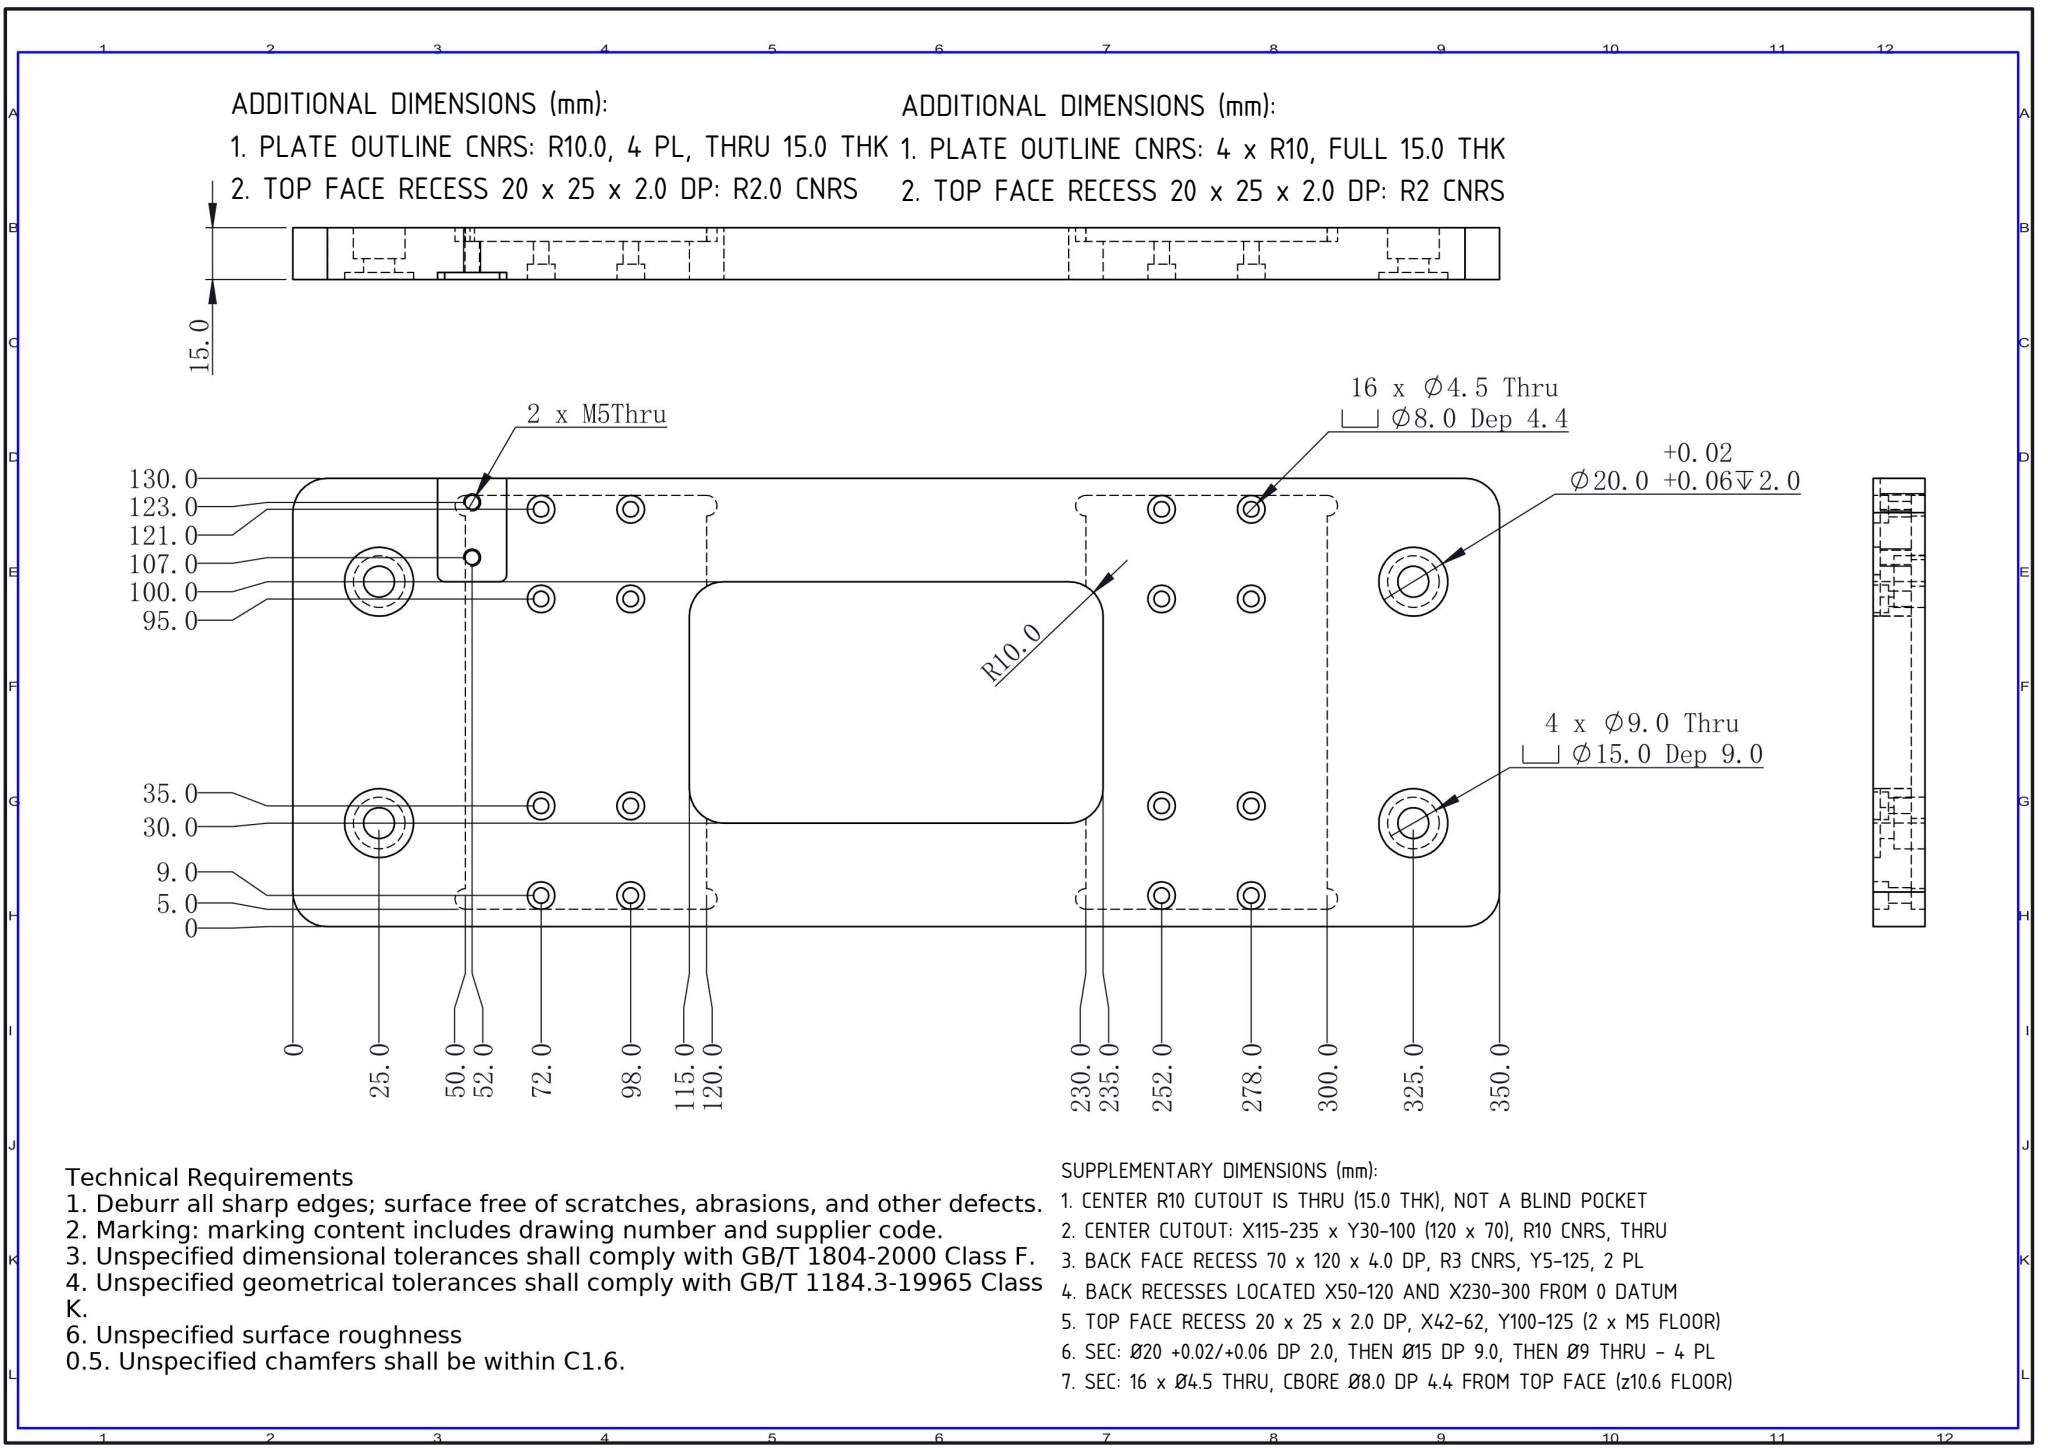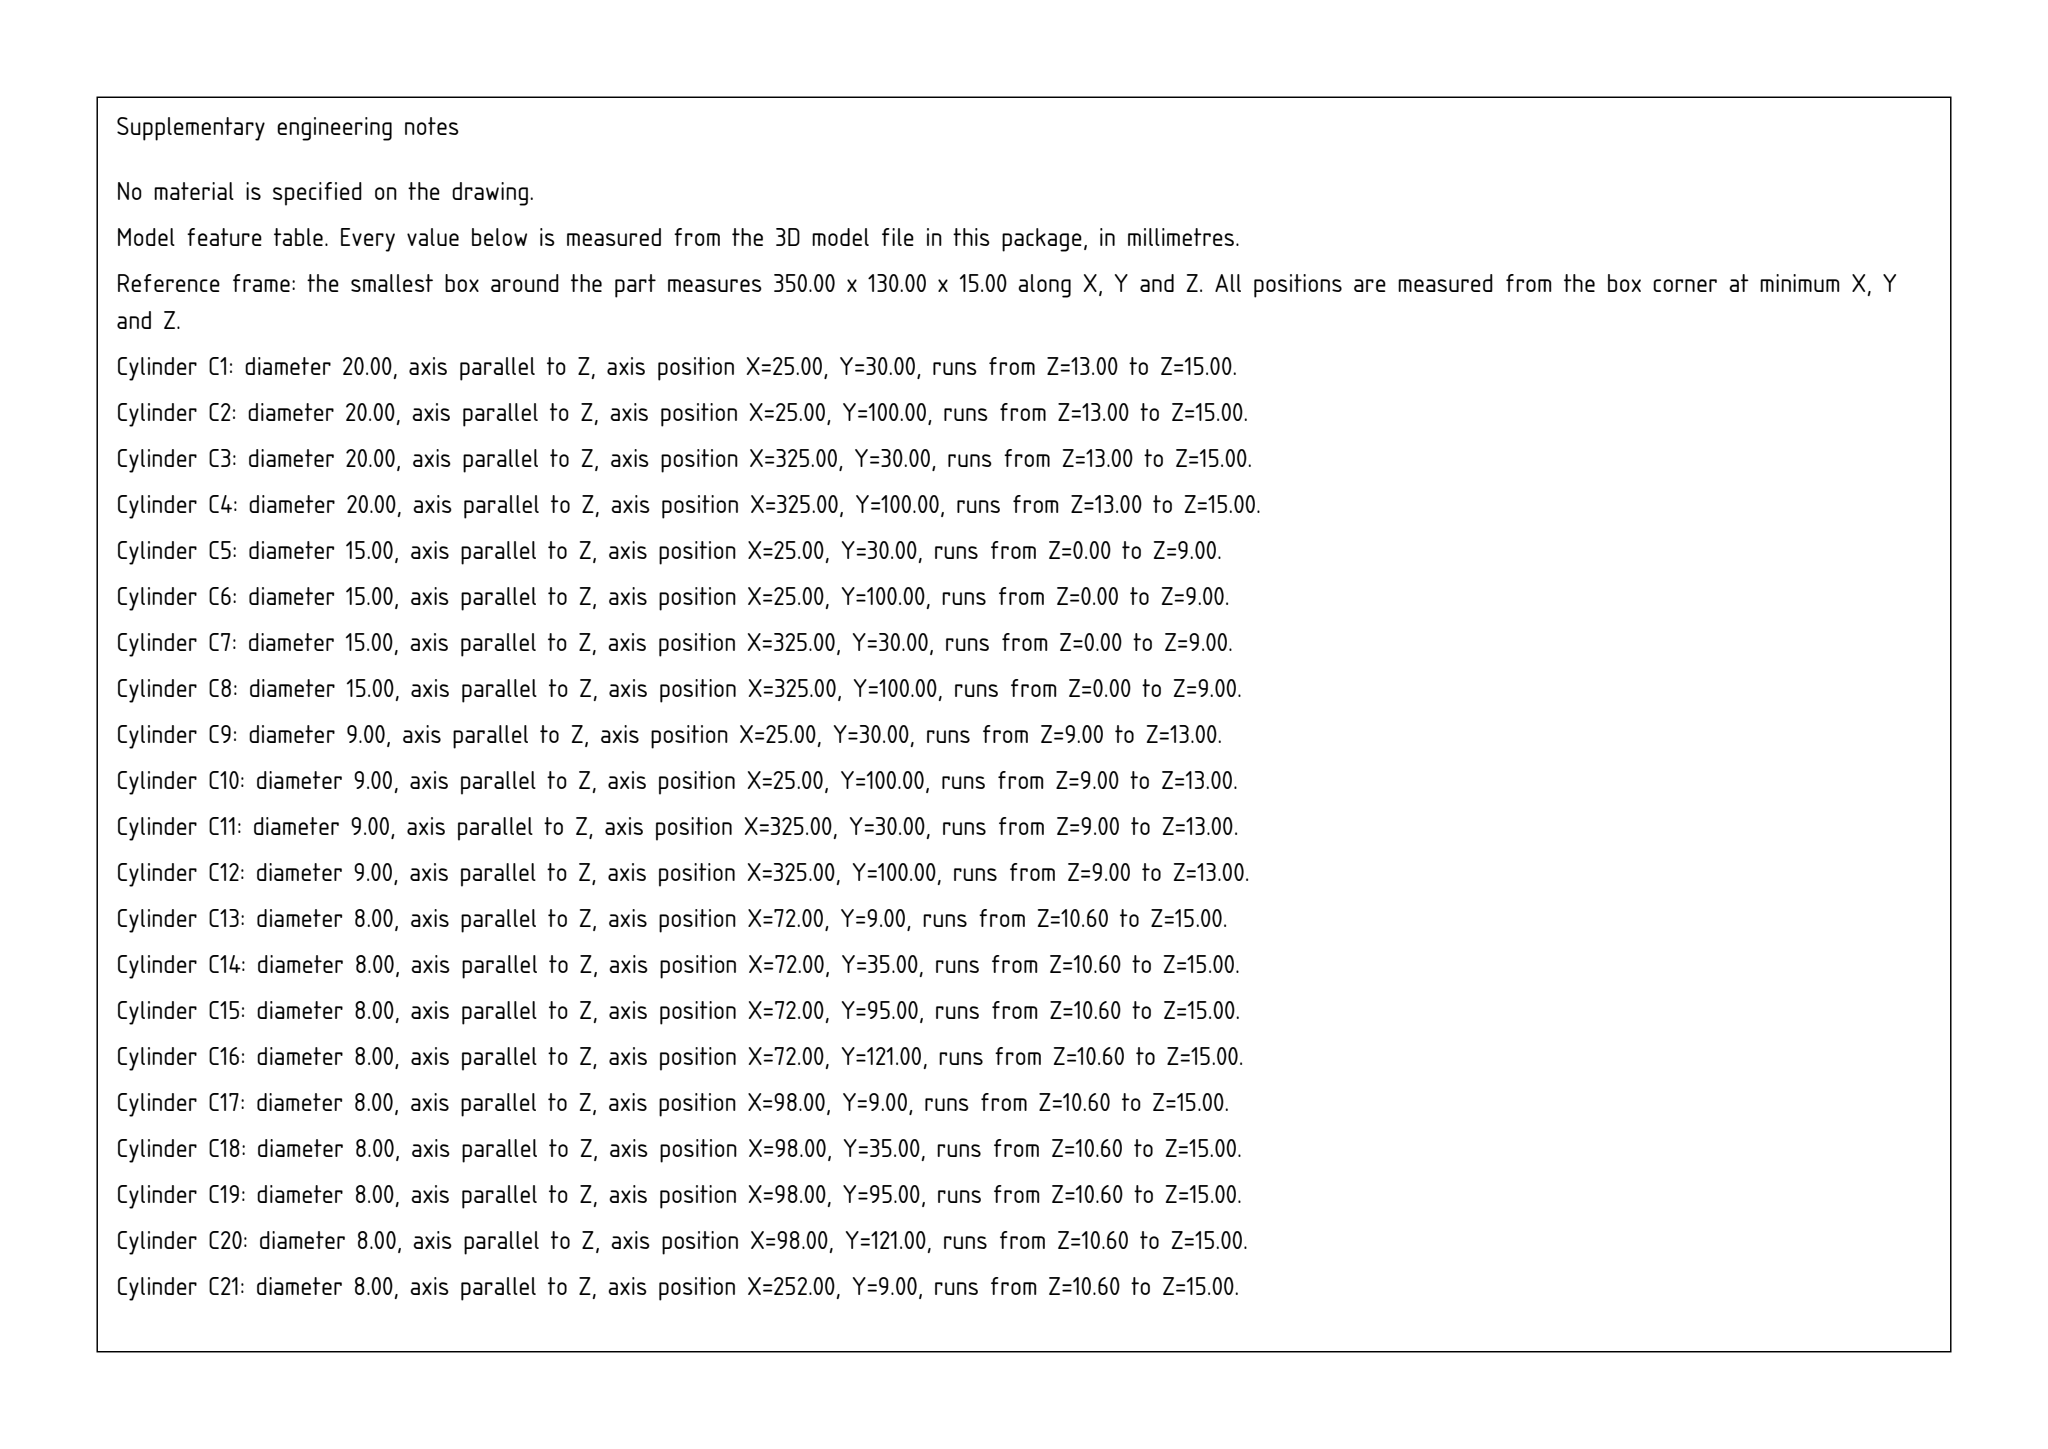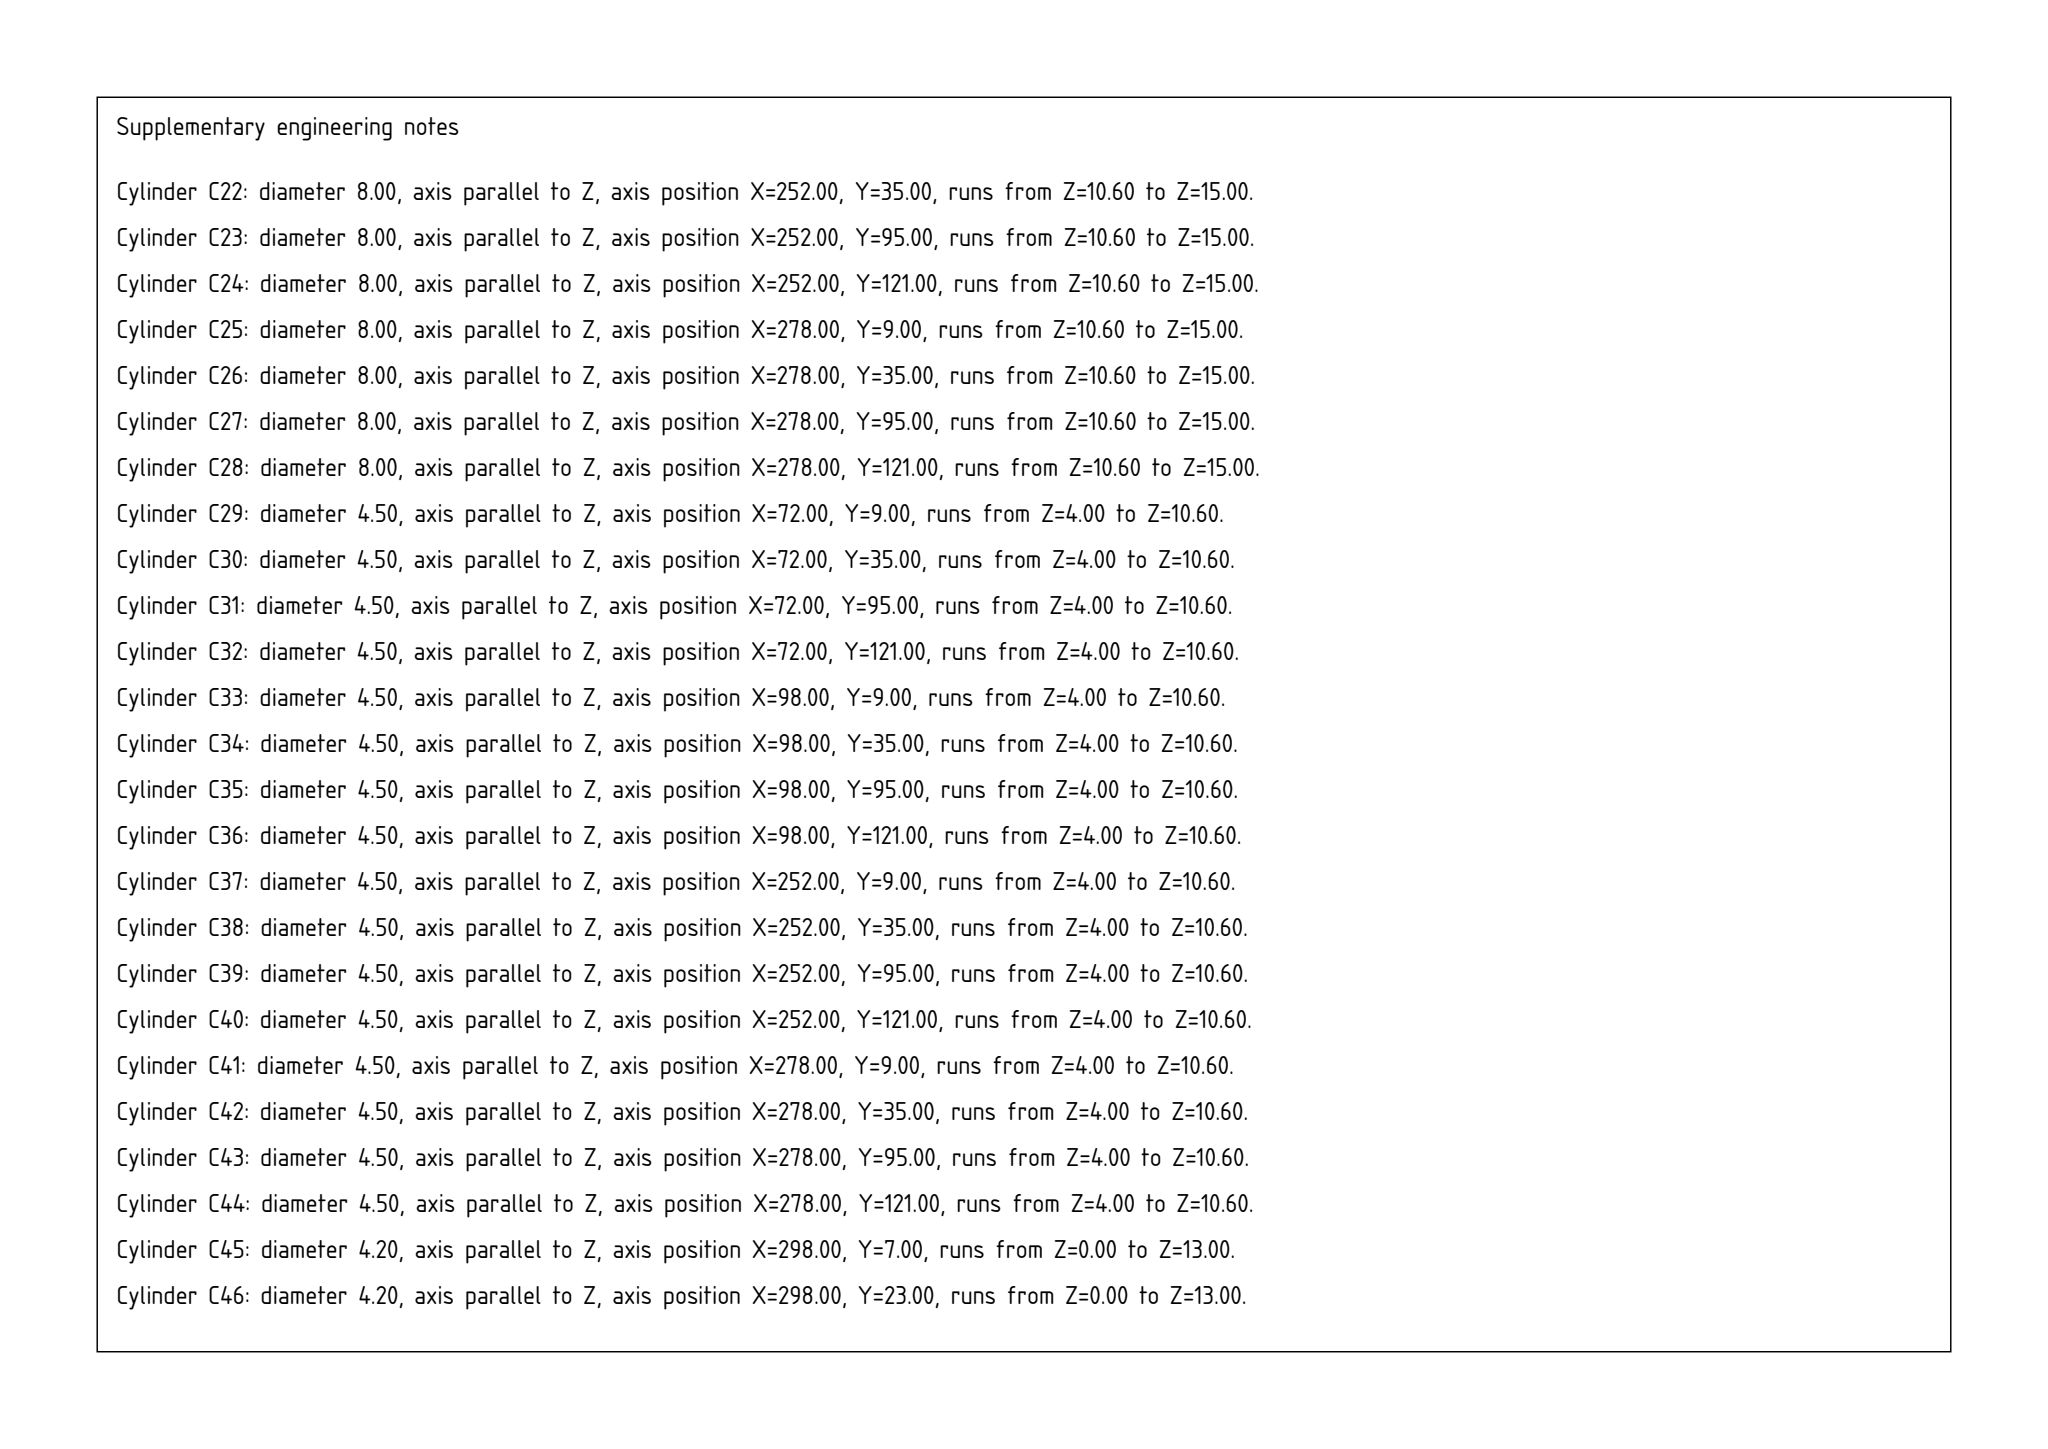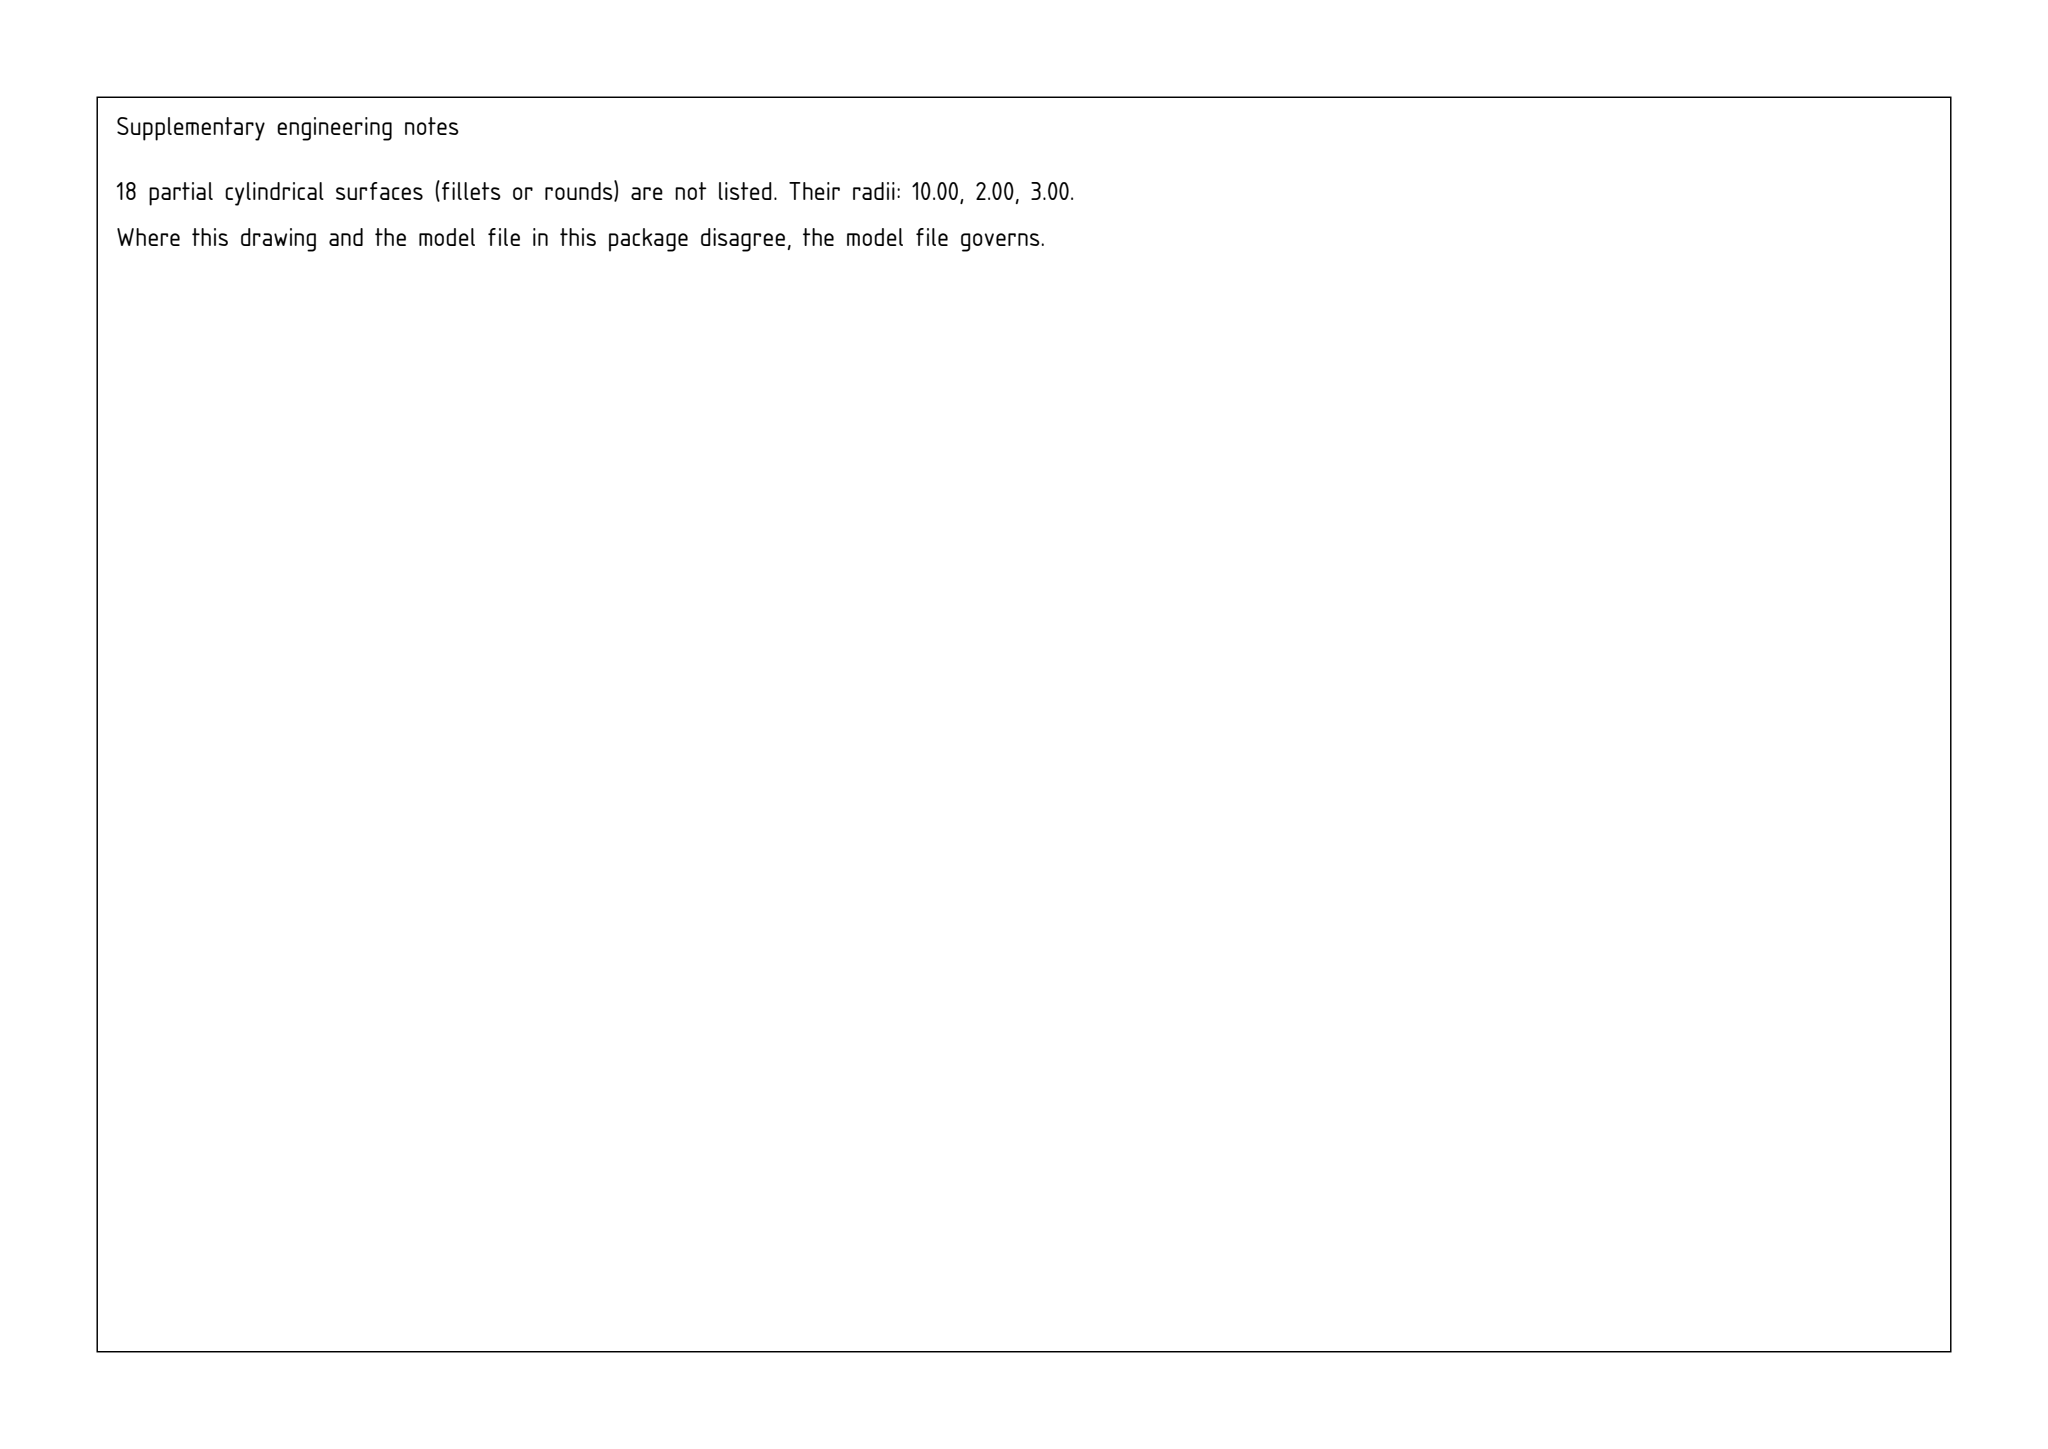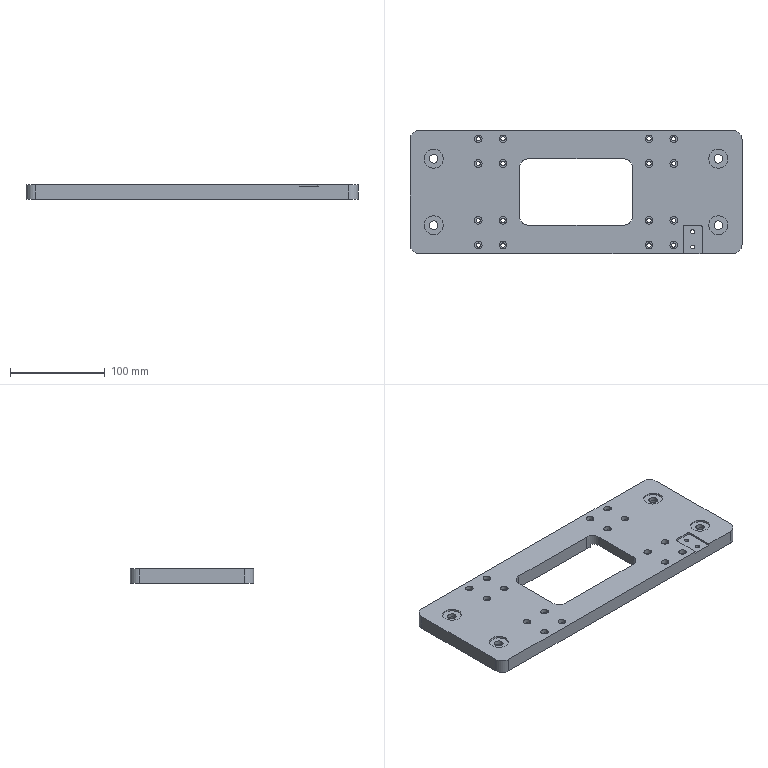Part | SolidWorks | mm | 1 solid | 166 faces | box 350 x 130 x 15 mm | volume 474781 mm3 | cylinder 114 | plane 52 | commonest cylinder face diameters 8 x32 4.5 x32 20 x16 6 x12 15 x8 9 x8 4.2 x4 4 x2
build123d program:
from build123d import *

# Parameters (mm, degrees)
SKETCH1_W                                       = 350
SKETCH1_H                                       = 130
BOSS_EXTRUDE1_DEPTH                             = 15
SKETCH2_R                                       = 10
CUT_EXTRUDE1_DEPTH                              = 2
FILLET1_R                                       = 10
M8_HEX_SOCKET_HEAD_CAP_SCREW_CBORE1_D           = 9
M8_HEX_SOCKET_HEAD_CAP_SCREW_CBORE1_CBORE_D     = 15
M8_HEX_SOCKET_HEAD_CAP_SCREW_CBORE1_CBORE_DEPTH = 9
SKETCH8_W                                       = 70
SKETCH8_H                                       = 120
CUT_EXTRUDE2_DEPTH                              = 4
SKETCH9_R                                       = 3
CUT_EXTRUDE4_DEPTH                              = 188.005
M4_HEX_SOCKET_HEAD_CAP_SCREW_CBORE1_D           = 4.5
M4_HEX_SOCKET_HEAD_CAP_SCREW_CBORE1_CBORE_D     = 8
M4_HEX_SOCKET_HEAD_CAP_SCREW_CBORE1_CBORE_DEPTH = 4.4
SKETCH12_W                                      = 120
SKETCH12_H                                      = 70
CUT_EXTRUDE5_DEPTH                              = 188.283
FILLET2_R                                       = 10
SKETCH13_W                                      = 20
SKETCH13_H                                      = 30
CUT_EXTRUDE6_DEPTH                              = 2
FILLET3_R                                       = 2
M5_TAPPED_HOLE1_D                               = 4.2


with BuildPart() as part:
    # Sketch1 → Boss-Extrude1 (new body)
    with BuildSketch(Plane.XY):
        Rectangle(SKETCH1_W, SKETCH1_H)
    extrude(amount=BOSS_EXTRUDE1_DEPTH)

    # Sketch2 → Cut-Extrude1 (cut)
    with BuildSketch(Plane.XY.offset(15)):
        with Locations((-150, 35)):
            Circle(SKETCH2_R)
        with Locations((-150, -35)):
            Circle(SKETCH2_R)
        with Locations((150, 35)):
            Circle(SKETCH2_R)
        with Locations((150, -35)):
            Circle(SKETCH2_R)
    extrude(amount=-CUT_EXTRUDE1_DEPTH, mode=Mode.SUBTRACT)

    # Fillet1
    fillet1_edges = [part.edges().sort_by_distance(p)[0] for p in [
        (175, -65, 7.5),
        (-175, -65, 7.5),
        (-175, 65, 7.5),
        (175, 65, 7.5),
    ]]
    fillet(fillet1_edges, radius=FILLET1_R)

    # M8 Hex Socket Head Cap Screw CBORE1 (through all)
    with Locations(Plane(origin=(0, 0, 0), x_dir=(-1, 0, 0), z_dir=(0, 0, -1))):
        with Locations((-150, -35), (-150, 35), (150, 35), (150, -35)):
            CounterBoreHole(M8_HEX_SOCKET_HEAD_CAP_SCREW_CBORE1_D / 2, M8_HEX_SOCKET_HEAD_CAP_SCREW_CBORE1_CBORE_D / 2, M8_HEX_SOCKET_HEAD_CAP_SCREW_CBORE1_CBORE_DEPTH)

    # Sketch8 → Cut-Extrude2 (cut)
    with BuildSketch(Plane(origin=(0, 0, 0), x_dir=(-1, 0, 0), z_dir=(0, 0, -1))):
        with Locations((-90, 0)):
            Rectangle(SKETCH8_W, SKETCH8_H)
        with Locations((90, 0)):
            Rectangle(SKETCH8_W, SKETCH8_H)
    extrude(amount=-CUT_EXTRUDE2_DEPTH, mode=Mode.SUBTRACT)

    # Sketch9 → Cut-Extrude4 (cut, through all)
    with BuildSketch(Plane(origin=(0, 0, 4), x_dir=(-1, 0, 0), z_dir=(0, 0, -1))):
        with Locations((-125, 57)):
            Circle(SKETCH9_R)
        with Locations((-55, 57)):
            Circle(SKETCH9_R)
        with Locations((-125, -57)):
            Circle(SKETCH9_R)
        with Locations((-55, -57)):
            Circle(SKETCH9_R)
        with Locations((55, -57)):
            Circle(SKETCH9_R)
        with Locations((125, -57)):
            Circle(SKETCH9_R)
        with Locations((55, 57)):
            Circle(SKETCH9_R)
        with Locations((125, 57)):
            Circle(SKETCH9_R)
    extrude(amount=CUT_EXTRUDE4_DEPTH, mode=Mode.SUBTRACT)

    # M4 Hex Socket Head Cap Screw CBORE1 (through all)
    with Locations(Plane.XY.offset(15)):
        with Locations((103, 30), (77, 30), (103, 56), (77, 56), (103, -56), (77, -56), (103, -30), (77, -30), (-77, -56), (-103, -56), (-77, -30), (-103, -30), (-77, 30), (-103, 30), (-77, 56), (-103, 56)):
            CounterBoreHole(M4_HEX_SOCKET_HEAD_CAP_SCREW_CBORE1_D / 2, M4_HEX_SOCKET_HEAD_CAP_SCREW_CBORE1_CBORE_D / 2, M4_HEX_SOCKET_HEAD_CAP_SCREW_CBORE1_CBORE_DEPTH)

    # Sketch12 → Cut-Extrude5 (cut, through all)
    with BuildSketch(Plane.XY.offset(15)):
        Rectangle(SKETCH12_W, SKETCH12_H)
    extrude(amount=-CUT_EXTRUDE5_DEPTH, mode=Mode.SUBTRACT)

    # Fillet2
    fillet2_edges = [part.edges().sort_by_distance(p)[0] for p in [
        (-60, -35, 9.5),
        (60, -35, 9.5),
        (60, 35, 9.5),
        (-60, 35, 9.5),
    ]]
    fillet(fillet2_edges, radius=FILLET2_R)

    # Sketch13 → Cut-Extrude6 (cut)
    with BuildSketch(Plane.XY.offset(15)):
        with Locations((123, -50)):
            Rectangle(SKETCH13_W, SKETCH13_H)
    extrude(amount=-CUT_EXTRUDE6_DEPTH, mode=Mode.SUBTRACT)

    # Fillet3
    fillet3_edges = [part.edges().sort_by_distance(p)[0] for p in [
        (133, -35, 14),
        (113, -35, 14),
    ]]
    fillet(fillet3_edges, radius=FILLET3_R)

    # M5 Tapped Hole1 (through all)
    with Locations(Plane.XY.offset(13)):
        with Locations((123, -42), (123, -58)):
            Hole(M5_TAPPED_HOLE1_D / 2)


solid = part.part